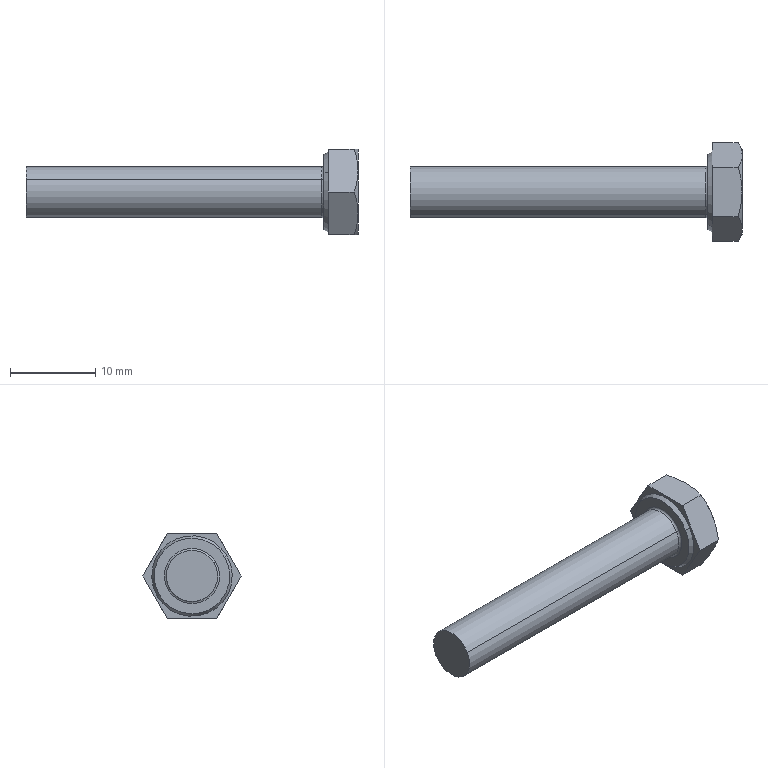Component | SolidWorks | GB_T5782-2016[HexHeadBoltM6_35]-4 | 1 solid | 22 faces | box 39 x 11.55 x 10 mm | volume 1325 mm3 | plane 10 | cone 8 | torus 2 | cylinder 2 | commonest cylinder face diameters 6 x2
build123d program:
from build123d import *

# Parameters (mm, degrees)
BASE_EXTRUDE_DEPTH = 4
FILLET_2_R         = 0.25


with BuildPart() as part:
    # Sketch1 → Base-Extrude (new body)
    with BuildSketch(Plane(origin=(0, 0, 0), x_dir=(0, 0, -1), z_dir=(1, 0, 0))):
        Polygon((5, 2.887), (5, -2.887), (0, -5.774), (-5, -2.887), (-5, 2.887), (0, 5.774), align=None)
    extrude(amount=BASE_EXTRUDE_DEPTH)

    # Sketch2 → Revolve1 (revolve)
    with BuildSketch(Plane.XY, mode=Mode.PRIVATE) as revolve1_sk:
        Polygon((0, 0), (39, 0), (39, 2.134), (39, 3), (21, 3), (0, 3), align=None)
    revolve(revolve1_sk.sketch.rotate(Axis((0, 0, 0), (1, 0, 0)), 90), axis=Axis((0, 0, 0), (1, 0, 0)))

    # Sketch3 → Cut-Revolve1 (revolve, cut)
    with BuildSketch(Plane.XY):
        Polygon((0, 5), (3.333, 10.774), (3.333, 15.774), (-10, 15.774), (-10, 5), align=None)
    revolve(axis=Axis((0, 0, 0), (1, 0, 0)), mode=Mode.SUBTRACT)

    # Sketch4 → Cut-Revolve3 (revolve, cut)
    with BuildSketch(Plane.XY, mode=Mode.PRIVATE) as cut_revolve3_sk:
        Polygon((4, 4.44), (3.5, 4.729), (3.5, 5.774), (4, 5.774), align=None)
    revolve(cut_revolve3_sk.sketch.rotate(Axis((0, 0, 0), (1, 0, 0)), 90), axis=Axis((0, 0, 0), (1, 0, 0)), mode=Mode.SUBTRACT)

    # Fillet 2
    fillet_2_edges = [part.edges().sort_by_distance(p)[0] for p in [
        (4, 0, -3),
    ]]
    fillet(fillet_2_edges, radius=FILLET_2_R)


solid = part.part

# Placed as in the assembly
solid = solid.moved(Location((4, 0, -95), (-180, 0, 180)))
STEP:
#1=COLOUR_RGB('',0.7922,0.8196,0.9333);
#2=FILL_AREA_STYLE_COLOUR('',#1);
#3=FILL_AREA_STYLE('',(#2));
#4=SURFACE_STYLE_FILL_AREA(#3);
#5=SURFACE_SIDE_STYLE('',(#4));
#6=SURFACE_STYLE_USAGE(.BOTH.,#5);
#7=PRESENTATION_STYLE_ASSIGNMENT((#6));
#8=CARTESIAN_POINT('',(-0.009843,-0.1023,-3.681));
#9=VERTEX_POINT('',#8);
#10=CARTESIAN_POINT('',(-0.009843,0.1023,-3.799));
#11=VERTEX_POINT('',#10);
#12=CARTESIAN_POINT('',(-0.009843,0.,-3.74));
#13=DIRECTION('',(-1.,-0.,0.));
#14=DIRECTION('',(-0.,0.866,-0.5));
#15=AXIS2_PLACEMENT_3D('',#12,#13,#14);
#16=CIRCLE('',#15,0.1181);
#17=EDGE_CURVE('',#9,#11,#16,.T.);
#18=ORIENTED_EDGE('',*,*,#17,.F.);
#19=CARTESIAN_POINT('',(0.,-0.1108,-3.676));
#20=VERTEX_POINT('',#19);
#21=CARTESIAN_POINT('',(-0.009843,-0.1108,-3.676));
#22=DIRECTION('',(0.,-0.5,-0.866));
#23=DIRECTION('',(0.,0.866,-0.5));
#24=AXIS2_PLACEMENT_3D('',#21,#22,#23);
#25=CIRCLE('',#24,0.009843);
#26=EDGE_CURVE('',#9,#20,#25,.T.);
#27=ORIENTED_EDGE('',*,*,#26,.T.);
#28=CARTESIAN_POINT('',(0.,0.1108,-3.804));
#29=VERTEX_POINT('',#28);
#30=CARTESIAN_POINT('',(0.,0.,-3.74));
#31=DIRECTION('',(1.,0.,-0.));
#32=DIRECTION('',(-0.,0.866,-0.5));
#33=AXIS2_PLACEMENT_3D('',#30,#31,#32);
#34=CIRCLE('',#33,0.128);
#35=EDGE_CURVE('',#29,#20,#34,.T.);
#36=ORIENTED_EDGE('',*,*,#35,.F.);
#37=CARTESIAN_POINT('',(-0.009843,0.1108,-3.804));
#38=DIRECTION('',(-0.,0.5,0.866));
#39=DIRECTION('',(0.,-0.866,0.5));
#40=AXIS2_PLACEMENT_3D('',#37,#38,#39);
#41=CIRCLE('',#40,0.009843);
#42=EDGE_CURVE('',#11,#29,#41,.T.);
#43=ORIENTED_EDGE('',*,*,#42,.F.);
#44=EDGE_LOOP('',(#18,#27,#36,#43));
#45=FACE_OUTER_BOUND('',#44,.T.);
#46=CARTESIAN_POINT('',(-0.009843,0.,-3.74));
#47=DIRECTION('',(-1.,-0.,0.));
#48=DIRECTION('',(-0.,0.866,-0.5));
#49=AXIS2_PLACEMENT_3D('',#46,#47,#48);
#50=TOROIDAL_SURFACE('',#49,0.128,0.009843);
#51=ADVANCED_FACE('',(#45),#50,.F.);
#52=CARTESIAN_POINT('',(-1.378,-0.1023,-3.681));
#53=VERTEX_POINT('',#52);
#54=CARTESIAN_POINT('',(-1.378,0.1023,-3.799));
#55=VERTEX_POINT('',#54);
#56=CARTESIAN_POINT('',(-1.378,0.,-3.74));
#57=DIRECTION('',(1.,0.,-0.));
#58=DIRECTION('',(0.,-0.866,0.5));
#59=AXIS2_PLACEMENT_3D('',#56,#57,#58);
#60=CIRCLE('',#59,0.1181);
#61=EDGE_CURVE('',#53,#55,#60,.T.);
#62=ORIENTED_EDGE('',*,*,#61,.T.);
#63=CARTESIAN_POINT('',(0.1575,0.1023,-3.799));
#64=DIRECTION('',(1.,0.,-0.));
#65=VECTOR('',#64,39.37);
#66=LINE('',#63,#65);
#67=EDGE_CURVE('',#55,#11,#66,.T.);
#68=ORIENTED_EDGE('',*,*,#67,.T.);
#69=CARTESIAN_POINT('',(-0.009843,0.,-3.74));
#70=DIRECTION('',(-1.,-0.,0.));
#71=DIRECTION('',(-0.,0.866,-0.5));
#72=AXIS2_PLACEMENT_3D('',#69,#70,#71);
#73=CIRCLE('',#72,0.1181);
#74=EDGE_CURVE('',#11,#9,#73,.T.);
#75=ORIENTED_EDGE('',*,*,#74,.T.);
#76=CARTESIAN_POINT('',(0.1575,-0.1023,-3.681));
#77=DIRECTION('',(1.,0.,-0.));
#78=VECTOR('',#77,39.37);
#79=LINE('',#76,#78);
#80=EDGE_CURVE('',#53,#9,#79,.T.);
#81=ORIENTED_EDGE('',*,*,#80,.F.);
#82=EDGE_LOOP('',(#62,#68,#75,#81));
#83=FACE_OUTER_BOUND('',#82,.T.);
#84=CARTESIAN_POINT('',(0.1575,0.,-3.74));
#85=DIRECTION('',(1.,0.,-0.));
#86=DIRECTION('',(0.,-0.866,0.5));
#87=AXIS2_PLACEMENT_3D('',#84,#85,#86);
#88=CYLINDRICAL_SURFACE('',#87,0.1181);
#89=ADVANCED_FACE('',(#83),#88,.T.);
#90=CARTESIAN_POINT('',(0.,-0.1514,-3.653));
#91=VERTEX_POINT('',#90);
#92=CARTESIAN_POINT('',(0.,0.1514,-3.828));
#93=VERTEX_POINT('',#92);
#94=CARTESIAN_POINT('',(0.,0.,-3.74));
#95=DIRECTION('',(1.,0.,-0.));
#96=DIRECTION('',(0.,-0.866,0.5));
#97=AXIS2_PLACEMENT_3D('',#94,#95,#96);
#98=CIRCLE('',#97,0.1748);
#99=EDGE_CURVE('',#91,#93,#98,.T.);
#100=ORIENTED_EDGE('',*,*,#99,.T.);
#101=CARTESIAN_POINT('',(0.01969,0.1612,-3.833));
#102=VERTEX_POINT('',#101);
#103=CARTESIAN_POINT('',(0.01969,0.1612,-3.833));
#104=DIRECTION('',(0.866,0.433,-0.25));
#105=VECTOR('',#104,39.37);
#106=LINE('',#103,#105);
#107=EDGE_CURVE('',#93,#102,#106,.T.);
#108=ORIENTED_EDGE('',*,*,#107,.T.);
#109=CARTESIAN_POINT('',(0.01969,-0.1612,-3.647));
#110=VERTEX_POINT('',#109);
#111=CARTESIAN_POINT('',(0.01969,0.,-3.74));
#112=DIRECTION('',(1.,0.,-0.));
#113=DIRECTION('',(0.,-0.866,0.5));
#114=AXIS2_PLACEMENT_3D('',#111,#112,#113);
#115=CIRCLE('',#114,0.1862);
#116=EDGE_CURVE('',#110,#102,#115,.T.);
#117=ORIENTED_EDGE('',*,*,#116,.F.);
#118=CARTESIAN_POINT('',(0.01969,-0.1612,-3.647));
#119=DIRECTION('',(0.866,-0.433,0.25));
#120=VECTOR('',#119,39.37);
#121=LINE('',#118,#120);
#122=EDGE_CURVE('',#91,#110,#121,.T.);
#123=ORIENTED_EDGE('',*,*,#122,.F.);
#124=EDGE_LOOP('',(#100,#108,#117,#123));
#125=FACE_OUTER_BOUND('',#124,.T.);
#126=CARTESIAN_POINT('',(0.01969,0.,-3.74));
#127=DIRECTION('',(1.,0.,-0.));
#128=DIRECTION('',(0.,-0.866,0.5));
#129=AXIS2_PLACEMENT_3D('',#126,#127,#128);
#130=CONICAL_SURFACE('',#129,0.1862,0.5236);
#131=ADVANCED_FACE('',(#125),#130,.T.);
#132=CARTESIAN_POINT('',(0.01969,0.1137,-3.937));
#133=VERTEX_POINT('',#132);
#134=CARTESIAN_POINT('',(0.01969,-0.1137,-3.937));
#135=VERTEX_POINT('',#134);
#136=CARTESIAN_POINT('',(0.01969,0.1137,-3.937));
#137=DIRECTION('',(0.,-1.,-0.));
#138=VECTOR('',#137,39.37);
#139=LINE('',#136,#138);
#140=EDGE_CURVE('',#133,#135,#139,.T.);
#141=ORIENTED_EDGE('',*,*,#140,.F.);
#142=CARTESIAN_POINT('',(0.1399,0.1137,-3.937));
#143=VERTEX_POINT('',#142);
#144=CARTESIAN_POINT('',(0.,0.1137,-3.937));
#145=DIRECTION('',(1.,0.,-0.));
#146=VECTOR('',#145,39.37);
#147=LINE('',#144,#146);
#148=EDGE_CURVE('',#133,#143,#147,.T.);
#149=ORIENTED_EDGE('',*,*,#148,.T.);
#150=CARTESIAN_POINT('',(0.1575,0.,-3.937));
#151=VERTEX_POINT('',#150);
#152=CARTESIAN_POINT('',(0.1575,0.,-3.937));
#153=CARTESIAN_POINT('',(0.1575,0.009645,-3.937));
#154=CARTESIAN_POINT('',(0.1571,0.01933,-3.937));
#155=CARTESIAN_POINT('',(0.1555,0.0385,-3.937));
#156=CARTESIAN_POINT('',(0.1543,0.04802,-3.937));
#157=CARTESIAN_POINT('',(0.1497,0.07641,-3.937));
#158=CARTESIAN_POINT('',(0.1453,0.09511,-3.937));
#159=CARTESIAN_POINT('',(0.1399,0.1137,-3.937));
#160=B_SPLINE_CURVE_WITH_KNOTS('',3,(#152,#153,#154,#155,#156,#157,#158,#159),.UNSPECIFIED.,.F.,.F.,(4,2,2,4),(0.002921,0.003649,0.004376,0.005831),.UNSPECIFIED.);
#161=EDGE_CURVE('',#151,#143,#160,.T.);
#162=ORIENTED_EDGE('',*,*,#161,.F.);
#163=CARTESIAN_POINT('',(0.1399,-0.1137,-3.937));
#164=VERTEX_POINT('',#163);
#165=CARTESIAN_POINT('',(0.1399,-0.1137,-3.937));
#166=CARTESIAN_POINT('',(0.1506,-0.07647,-3.937));
#167=CARTESIAN_POINT('',(0.1575,-0.03873,-3.937));
#168=CARTESIAN_POINT('',(0.1575,0.,-3.937));
#169=B_SPLINE_CURVE_WITH_KNOTS('',3,(#165,#166,#167,#168),.UNSPECIFIED.,.F.,.F.,(4,4),(0.00000024,0.002921),.UNSPECIFIED.);
#170=EDGE_CURVE('',#164,#151,#169,.T.);
#171=ORIENTED_EDGE('',*,*,#170,.F.);
#172=CARTESIAN_POINT('',(0.,-0.1137,-3.937));
#173=DIRECTION('',(1.,0.,-0.));
#174=VECTOR('',#173,39.37);
#175=LINE('',#172,#174);
#176=EDGE_CURVE('',#135,#164,#175,.T.);
#177=ORIENTED_EDGE('',*,*,#176,.F.);
#178=EDGE_LOOP('',(#141,#149,#162,#171,#177));
#179=FACE_OUTER_BOUND('',#178,.T.);
#180=CARTESIAN_POINT('',(0.,0.1137,-3.937));
#181=DIRECTION('',(0.,-0.,1.));
#182=DIRECTION('',(-0.,1.,0.));
#183=AXIS2_PLACEMENT_3D('',#180,#181,#182);
#184=PLANE('',#183);
#185=ADVANCED_FACE('',(#179),#184,.F.);
#186=CARTESIAN_POINT('',(0.01969,-0.2273,-3.74));
#187=VERTEX_POINT('',#186);
#188=CARTESIAN_POINT('',(0.01969,-0.1137,-3.937));
#189=DIRECTION('',(0.,-0.5,0.866));
#190=VECTOR('',#189,39.37);
#191=LINE('',#188,#190);
#192=EDGE_CURVE('',#135,#187,#191,.T.);
#193=ORIENTED_EDGE('',*,*,#192,.F.);
#194=ORIENTED_EDGE('',*,*,#176,.T.);
#195=CARTESIAN_POINT('',(0.1575,-0.1705,-3.839));
#196=VERTEX_POINT('',#195);
#197=CARTESIAN_POINT('',(0.1575,-0.1705,-3.839));
#198=CARTESIAN_POINT('',(0.1575,-0.1657,-3.847));
#199=CARTESIAN_POINT('',(0.1571,-0.1608,-3.855));
#200=CARTESIAN_POINT('',(0.1555,-0.1512,-3.872));
#201=CARTESIAN_POINT('',(0.1543,-0.1465,-3.88));
#202=CARTESIAN_POINT('',(0.1497,-0.1323,-3.905));
#203=CARTESIAN_POINT('',(0.1453,-0.1229,-3.921));
#204=CARTESIAN_POINT('',(0.1399,-0.1137,-3.937));
#205=B_SPLINE_CURVE_WITH_KNOTS('',3,(#197,#198,#199,#200,#201,#202,#203,#204),.UNSPECIFIED.,.F.,.F.,(4,2,2,4),(0.002921,0.003649,0.004376,0.005831),.UNSPECIFIED.);
#206=EDGE_CURVE('',#196,#164,#205,.T.);
#207=ORIENTED_EDGE('',*,*,#206,.F.);
#208=CARTESIAN_POINT('',(0.1399,-0.2273,-3.74));
#209=VERTEX_POINT('',#208);
#210=CARTESIAN_POINT('',(0.1399,-0.2273,-3.74));
#211=CARTESIAN_POINT('',(0.1506,-0.2087,-3.772));
#212=CARTESIAN_POINT('',(0.1575,-0.1898,-3.805));
#213=CARTESIAN_POINT('',(0.1575,-0.1705,-3.839));
#214=B_SPLINE_CURVE_WITH_KNOTS('',3,(#210,#211,#212,#213),.UNSPECIFIED.,.F.,.F.,(4,4),(0.00000024,0.002921),.UNSPECIFIED.);
#215=EDGE_CURVE('',#209,#196,#214,.T.);
#216=ORIENTED_EDGE('',*,*,#215,.F.);
#217=CARTESIAN_POINT('',(0.,-0.2273,-3.74));
#218=DIRECTION('',(1.,0.,-0.));
#219=VECTOR('',#218,39.37);
#220=LINE('',#217,#219);
#221=EDGE_CURVE('',#187,#209,#220,.T.);
#222=ORIENTED_EDGE('',*,*,#221,.F.);
#223=EDGE_LOOP('',(#193,#194,#207,#216,#222));
#224=FACE_OUTER_BOUND('',#223,.T.);
#225=CARTESIAN_POINT('',(0.,-0.1137,-3.937));
#226=DIRECTION('',(-0.,0.866,0.5));
#227=DIRECTION('',(-0.,0.5,-0.866));
#228=AXIS2_PLACEMENT_3D('',#225,#226,#227);
#229=PLANE('',#228);
#230=ADVANCED_FACE('',(#224),#229,.F.);
#231=CARTESIAN_POINT('',(0.01969,-0.1137,-3.543));
#232=VERTEX_POINT('',#231);
#233=CARTESIAN_POINT('',(0.01969,-0.2273,-3.74));
#234=DIRECTION('',(-0.,0.5,0.866));
#235=VECTOR('',#234,39.37);
#236=LINE('',#233,#235);
#237=EDGE_CURVE('',#187,#232,#236,.T.);
#238=ORIENTED_EDGE('',*,*,#237,.F.);
#239=ORIENTED_EDGE('',*,*,#221,.T.);
#240=CARTESIAN_POINT('',(0.1575,-0.1705,-3.642));
#241=VERTEX_POINT('',#240);
#242=CARTESIAN_POINT('',(0.1575,-0.1705,-3.642));
#243=CARTESIAN_POINT('',(0.1575,-0.1801,-3.658));
#244=CARTESIAN_POINT('',(0.1558,-0.1898,-3.675));
#245=CARTESIAN_POINT('',(0.1496,-0.2088,-3.708));
#246=CARTESIAN_POINT('',(0.1452,-0.2181,-3.724));
#247=CARTESIAN_POINT('',(0.1399,-0.2273,-3.74));
#248=B_SPLINE_CURVE_WITH_KNOTS('',3,(#242,#243,#244,#245,#246,#247),.UNSPECIFIED.,.F.,.F.,(4,2,4),(0.008262,0.009724,0.01119),.UNSPECIFIED.);
#249=EDGE_CURVE('',#241,#209,#248,.T.);
#250=ORIENTED_EDGE('',*,*,#249,.F.);
#251=CARTESIAN_POINT('',(0.1399,-0.1137,-3.543));
#252=VERTEX_POINT('',#251);
#253=CARTESIAN_POINT('',(0.1399,-0.1137,-3.543));
#254=CARTESIAN_POINT('',(0.1452,-0.1229,-3.559));
#255=CARTESIAN_POINT('',(0.1497,-0.1324,-3.576));
#256=CARTESIAN_POINT('',(0.1558,-0.1513,-3.609));
#257=CARTESIAN_POINT('',(0.1575,-0.1609,-3.625));
#258=CARTESIAN_POINT('',(0.1575,-0.1705,-3.642));
#259=B_SPLINE_CURVE_WITH_KNOTS('',3,(#253,#254,#255,#256,#257,#258),.UNSPECIFIED.,.F.,.F.,(4,2,4),(0.00534,0.006801,0.008262),.UNSPECIFIED.);
#260=EDGE_CURVE('',#252,#241,#259,.T.);
#261=ORIENTED_EDGE('',*,*,#260,.F.);
#262=CARTESIAN_POINT('',(0.,-0.1137,-3.543));
#263=DIRECTION('',(1.,0.,-0.));
#264=VECTOR('',#263,39.37);
#265=LINE('',#262,#264);
#266=EDGE_CURVE('',#232,#252,#265,.T.);
#267=ORIENTED_EDGE('',*,*,#266,.F.);
#268=EDGE_LOOP('',(#238,#239,#250,#261,#267));
#269=FACE_OUTER_BOUND('',#268,.T.);
#270=CARTESIAN_POINT('',(0.,-0.2273,-3.74));
#271=DIRECTION('',(-0.,0.866,-0.5));
#272=DIRECTION('',(1.,0.,-0.));
#273=AXIS2_PLACEMENT_3D('',#270,#271,#272);
#274=PLANE('',#273);
#275=ADVANCED_FACE('',(#269),#274,.F.);
#276=CARTESIAN_POINT('',(0.01969,0.1137,-3.543));
#277=VERTEX_POINT('',#276);
#278=CARTESIAN_POINT('',(0.01969,0.1137,-3.543));
#279=DIRECTION('',(-0.,1.,0.));
#280=VECTOR('',#279,39.37);
#281=LINE('',#278,#280);
#282=EDGE_CURVE('',#232,#277,#281,.T.);
#283=ORIENTED_EDGE('',*,*,#282,.F.);
#284=ORIENTED_EDGE('',*,*,#266,.T.);
#285=CARTESIAN_POINT('',(0.1575,0.,-3.543));
#286=VERTEX_POINT('',#285);
#287=CARTESIAN_POINT('',(0.1575,0.,-3.543));
#288=CARTESIAN_POINT('',(0.1575,-0.009645,-3.543));
#289=CARTESIAN_POINT('',(0.1571,-0.01933,-3.543));
#290=CARTESIAN_POINT('',(0.1555,-0.0385,-3.543));
#291=CARTESIAN_POINT('',(0.1543,-0.04802,-3.543));
#292=CARTESIAN_POINT('',(0.1497,-0.07641,-3.543));
#293=CARTESIAN_POINT('',(0.1453,-0.09511,-3.543));
#294=CARTESIAN_POINT('',(0.1399,-0.1137,-3.543));
#295=B_SPLINE_CURVE_WITH_KNOTS('',3,(#287,#288,#289,#290,#291,#292,#293,#294),.UNSPECIFIED.,.F.,.F.,(4,2,2,4),(0.002921,0.003649,0.004376,0.005831),.UNSPECIFIED.);
#296=EDGE_CURVE('',#286,#252,#295,.T.);
#297=ORIENTED_EDGE('',*,*,#296,.F.);
#298=CARTESIAN_POINT('',(0.1399,0.1137,-3.543));
#299=VERTEX_POINT('',#298);
#300=CARTESIAN_POINT('',(0.1399,0.1137,-3.543));
#301=CARTESIAN_POINT('',(0.1506,0.07647,-3.543));
#302=CARTESIAN_POINT('',(0.1575,0.03873,-3.543));
#303=CARTESIAN_POINT('',(0.1575,0.,-3.543));
#304=B_SPLINE_CURVE_WITH_KNOTS('',3,(#300,#301,#302,#303),.UNSPECIFIED.,.F.,.F.,(4,4),(0.00000024,0.002921),.UNSPECIFIED.);
#305=EDGE_CURVE('',#299,#286,#304,.T.);
#306=ORIENTED_EDGE('',*,*,#305,.F.);
#307=CARTESIAN_POINT('',(0.,0.1137,-3.543));
#308=DIRECTION('',(1.,0.,-0.));
#309=VECTOR('',#308,39.37);
#310=LINE('',#307,#309);
#311=EDGE_CURVE('',#277,#299,#310,.T.);
#312=ORIENTED_EDGE('',*,*,#311,.F.);
#313=EDGE_LOOP('',(#283,#284,#297,#306,#312));
#314=FACE_OUTER_BOUND('',#313,.T.);
#315=CARTESIAN_POINT('',(0.,0.1137,-3.543));
#316=DIRECTION('',(-0.,0.,-1.));
#317=DIRECTION('',(0.,-1.,-0.));
#318=AXIS2_PLACEMENT_3D('',#315,#316,#317);
#319=PLANE('',#318);
#320=ADVANCED_FACE('',(#314),#319,.F.);
#321=CARTESIAN_POINT('',(0.01969,0.2273,-3.74));
#322=VERTEX_POINT('',#321);
#323=CARTESIAN_POINT('',(0.01969,0.2273,-3.74));
#324=DIRECTION('',(-0.,0.5,-0.866));
#325=VECTOR('',#324,39.37);
#326=LINE('',#323,#325);
#327=EDGE_CURVE('',#277,#322,#326,.T.);
#328=ORIENTED_EDGE('',*,*,#327,.F.);
#329=ORIENTED_EDGE('',*,*,#311,.T.);
#330=CARTESIAN_POINT('',(0.1575,0.1705,-3.642));
#331=VERTEX_POINT('',#330);
#332=CARTESIAN_POINT('',(0.1575,0.1705,-3.642));
#333=CARTESIAN_POINT('',(0.1575,0.1657,-3.633));
#334=CARTESIAN_POINT('',(0.1571,0.1608,-3.625));
#335=CARTESIAN_POINT('',(0.1555,0.1512,-3.608));
#336=CARTESIAN_POINT('',(0.1543,0.1465,-3.6));
#337=CARTESIAN_POINT('',(0.1497,0.1323,-3.576));
#338=CARTESIAN_POINT('',(0.1453,0.1229,-3.559));
#339=CARTESIAN_POINT('',(0.1399,0.1137,-3.543));
#340=B_SPLINE_CURVE_WITH_KNOTS('',3,(#332,#333,#334,#335,#336,#337,#338,#339),.UNSPECIFIED.,.F.,.F.,(4,2,2,4),(0.002921,0.003649,0.004376,0.005831),.UNSPECIFIED.);
#341=EDGE_CURVE('',#331,#299,#340,.T.);
#342=ORIENTED_EDGE('',*,*,#341,.F.);
#343=CARTESIAN_POINT('',(0.1399,0.2273,-3.74));
#344=VERTEX_POINT('',#343);
#345=CARTESIAN_POINT('',(0.1399,0.2273,-3.74));
#346=CARTESIAN_POINT('',(0.1506,0.2087,-3.708));
#347=CARTESIAN_POINT('',(0.1575,0.1898,-3.675));
#348=CARTESIAN_POINT('',(0.1575,0.1705,-3.642));
#349=B_SPLINE_CURVE_WITH_KNOTS('',3,(#345,#346,#347,#348),.UNSPECIFIED.,.F.,.F.,(4,4),(0.00000024,0.002921),.UNSPECIFIED.);
#350=EDGE_CURVE('',#344,#331,#349,.T.);
#351=ORIENTED_EDGE('',*,*,#350,.F.);
#352=CARTESIAN_POINT('',(0.,0.2273,-3.74));
#353=DIRECTION('',(1.,0.,-0.));
#354=VECTOR('',#353,39.37);
#355=LINE('',#352,#354);
#356=EDGE_CURVE('',#322,#344,#355,.T.);
#357=ORIENTED_EDGE('',*,*,#356,.F.);
#358=EDGE_LOOP('',(#328,#329,#342,#351,#357));
#359=FACE_OUTER_BOUND('',#358,.T.);
#360=CARTESIAN_POINT('',(0.,0.2273,-3.74));
#361=DIRECTION('',(0.,-0.866,-0.5));
#362=DIRECTION('',(0.,-0.5,0.866));
#363=AXIS2_PLACEMENT_3D('',#360,#361,#362);
#364=PLANE('',#363);
#365=ADVANCED_FACE('',(#359),#364,.F.);
#366=CARTESIAN_POINT('',(0.01969,0.1137,-3.937));
#367=DIRECTION('',(0.,-0.5,-0.866));
#368=VECTOR('',#367,39.37);
#369=LINE('',#366,#368);
#370=EDGE_CURVE('',#322,#133,#369,.T.);
#371=ORIENTED_EDGE('',*,*,#370,.F.);
#372=ORIENTED_EDGE('',*,*,#356,.T.);
#373=CARTESIAN_POINT('',(0.1575,0.1705,-3.839));
#374=VERTEX_POINT('',#373);
#375=CARTESIAN_POINT('',(0.1575,0.1705,-3.839));
#376=CARTESIAN_POINT('',(0.1575,0.1801,-3.822));
#377=CARTESIAN_POINT('',(0.1558,0.1896,-3.805));
#378=CARTESIAN_POINT('',(0.1497,0.2086,-3.773));
#379=CARTESIAN_POINT('',(0.1452,0.2181,-3.756));
#380=CARTESIAN_POINT('',(0.1399,0.2273,-3.74));
#381=B_SPLINE_CURVE_WITH_KNOTS('',3,(#375,#376,#377,#378,#379,#380),.UNSPECIFIED.,.F.,.F.,(4,2,4),(0.01799,0.01945,0.02091),.UNSPECIFIED.);
#382=EDGE_CURVE('',#374,#344,#381,.T.);
#383=ORIENTED_EDGE('',*,*,#382,.F.);
#384=CARTESIAN_POINT('',(0.1399,0.1137,-3.937));
#385=CARTESIAN_POINT('',(0.1452,0.1228,-3.921));
#386=CARTESIAN_POINT('',(0.1496,0.1322,-3.905));
#387=CARTESIAN_POINT('',(0.1558,0.1511,-3.872));
#388=CARTESIAN_POINT('',(0.1575,0.1609,-3.855));
#389=CARTESIAN_POINT('',(0.1575,0.1705,-3.839));
#390=B_SPLINE_CURVE_WITH_KNOTS('',3,(#384,#385,#386,#387,#388,#389),.UNSPECIFIED.,.F.,.F.,(4,2,4),(0.01507,0.01653,0.01799),.UNSPECIFIED.);
#391=EDGE_CURVE('',#143,#374,#390,.T.);
#392=ORIENTED_EDGE('',*,*,#391,.F.);
#393=ORIENTED_EDGE('',*,*,#148,.F.);
#394=EDGE_LOOP('',(#371,#372,#383,#392,#393));
#395=FACE_OUTER_BOUND('',#394,.T.);
#396=CARTESIAN_POINT('',(0.,0.1137,-3.937));
#397=DIRECTION('',(0.,-0.866,0.5));
#398=DIRECTION('',(-0.,0.5,0.866));
#399=AXIS2_PLACEMENT_3D('',#396,#397,#398);
#400=PLANE('',#399);
#401=ADVANCED_FACE('',(#395),#400,.F.);
#402=ORIENTED_EDGE('',*,*,#350,.T.);
#403=CARTESIAN_POINT('',(0.1575,0.,-3.74));
#404=DIRECTION('',(-1.,-0.,0.));
#405=DIRECTION('',(-0.,0.866,-0.5));
#406=AXIS2_PLACEMENT_3D('',#403,#404,#405);
#407=CIRCLE('',#406,0.1969);
#408=EDGE_CURVE('',#331,#374,#407,.T.);
#409=ORIENTED_EDGE('',*,*,#408,.T.);
#410=ORIENTED_EDGE('',*,*,#382,.T.);
#411=EDGE_LOOP('',(#402,#409,#410));
#412=FACE_OUTER_BOUND('',#411,.T.);
#413=CARTESIAN_POINT('',(0.1575,0.,-3.74));
#414=DIRECTION('',(-1.,-0.,0.));
#415=DIRECTION('',(-0.,0.866,-0.5));
#416=AXIS2_PLACEMENT_3D('',#413,#414,#415);
#417=CONICAL_SURFACE('',#416,0.1969,1.047);
#418=ADVANCED_FACE('',(#412),#417,.T.);
#419=ORIENTED_EDGE('',*,*,#305,.T.);
#420=CARTESIAN_POINT('',(0.1575,0.,-3.74));
#421=DIRECTION('',(-1.,-0.,0.));
#422=DIRECTION('',(-0.,0.866,-0.5));
#423=AXIS2_PLACEMENT_3D('',#420,#421,#422);
#424=CIRCLE('',#423,0.1969);
#425=EDGE_CURVE('',#286,#331,#424,.T.);
#426=ORIENTED_EDGE('',*,*,#425,.T.);
#427=ORIENTED_EDGE('',*,*,#341,.T.);
#428=EDGE_LOOP('',(#419,#426,#427));
#429=FACE_OUTER_BOUND('',#428,.T.);
#430=CARTESIAN_POINT('',(0.1575,0.,-3.74));
#431=DIRECTION('',(-1.,-0.,0.));
#432=DIRECTION('',(-0.,0.866,-0.5));
#433=AXIS2_PLACEMENT_3D('',#430,#431,#432);
#434=CONICAL_SURFACE('',#433,0.1969,1.047);
#435=ADVANCED_FACE('',(#429),#434,.T.);
#436=ORIENTED_EDGE('',*,*,#260,.T.);
#437=CARTESIAN_POINT('',(0.1575,0.,-3.74));
#438=DIRECTION('',(-1.,-0.,0.));
#439=DIRECTION('',(-0.,0.866,-0.5));
#440=AXIS2_PLACEMENT_3D('',#437,#438,#439);
#441=CIRCLE('',#440,0.1969);
#442=EDGE_CURVE('',#241,#286,#441,.T.);
#443=ORIENTED_EDGE('',*,*,#442,.T.);
#444=ORIENTED_EDGE('',*,*,#296,.T.);
#445=EDGE_LOOP('',(#436,#443,#444));
#446=FACE_OUTER_BOUND('',#445,.T.);
#447=CARTESIAN_POINT('',(0.1575,0.,-3.74));
#448=DIRECTION('',(-1.,-0.,0.));
#449=DIRECTION('',(-0.,0.866,-0.5));
#450=AXIS2_PLACEMENT_3D('',#447,#448,#449);
#451=CONICAL_SURFACE('',#450,0.1969,1.047);
#452=ADVANCED_FACE('',(#446),#451,.T.);
#453=ORIENTED_EDGE('',*,*,#249,.T.);
#454=ORIENTED_EDGE('',*,*,#215,.T.);
#455=CARTESIAN_POINT('',(0.1575,0.,-3.74));
#456=DIRECTION('',(1.,0.,-0.));
#457=DIRECTION('',(0.,-0.866,0.5));
#458=AXIS2_PLACEMENT_3D('',#455,#456,#457);
#459=CIRCLE('',#458,0.1969);
#460=EDGE_CURVE('',#241,#196,#459,.T.);
#461=ORIENTED_EDGE('',*,*,#460,.F.);
#462=EDGE_LOOP('',(#453,#454,#461));
#463=FACE_OUTER_BOUND('',#462,.T.);
#464=CARTESIAN_POINT('',(0.1575,0.,-3.74));
#465=DIRECTION('',(-1.,-0.,0.));
#466=DIRECTION('',(-0.,0.866,-0.5));
#467=AXIS2_PLACEMENT_3D('',#464,#465,#466);
#468=CONICAL_SURFACE('',#467,0.1969,1.047);
#469=ADVANCED_FACE('',(#463),#468,.T.);
#470=ORIENTED_EDGE('',*,*,#206,.T.);
#471=ORIENTED_EDGE('',*,*,#170,.T.);
#472=CARTESIAN_POINT('',(0.1575,0.,-3.74));
#473=DIRECTION('',(-1.,-0.,0.));
#474=DIRECTION('',(-0.,0.866,-0.5));
#475=AXIS2_PLACEMENT_3D('',#472,#473,#474);
#476=CIRCLE('',#475,0.1969);
#477=EDGE_CURVE('',#151,#196,#476,.T.);
#478=ORIENTED_EDGE('',*,*,#477,.T.);
#479=EDGE_LOOP('',(#470,#471,#478));
#480=FACE_OUTER_BOUND('',#479,.T.);
#481=CARTESIAN_POINT('',(0.1575,0.,-3.74));
#482=DIRECTION('',(-1.,-0.,0.));
#483=DIRECTION('',(-0.,0.866,-0.5));
#484=AXIS2_PLACEMENT_3D('',#481,#482,#483);
#485=CONICAL_SURFACE('',#484,0.1969,1.047);
#486=ADVANCED_FACE('',(#480),#485,.T.);
#487=ORIENTED_EDGE('',*,*,#161,.T.);
#488=ORIENTED_EDGE('',*,*,#391,.T.);
#489=CARTESIAN_POINT('',(0.1575,0.,-3.74));
#490=DIRECTION('',(-1.,-0.,0.));
#491=DIRECTION('',(-0.,0.866,-0.5));
#492=AXIS2_PLACEMENT_3D('',#489,#490,#491);
#493=CIRCLE('',#492,0.1969);
#494=EDGE_CURVE('',#374,#151,#493,.T.);
#495=ORIENTED_EDGE('',*,*,#494,.T.);
#496=EDGE_LOOP('',(#487,#488,#495));
#497=FACE_OUTER_BOUND('',#496,.T.);
#498=CARTESIAN_POINT('',(0.1575,0.,-3.74));
#499=DIRECTION('',(-1.,-0.,0.));
#500=DIRECTION('',(-0.,0.866,-0.5));
#501=AXIS2_PLACEMENT_3D('',#498,#499,#500);
#502=CONICAL_SURFACE('',#501,0.1969,1.047);
#503=ADVANCED_FACE('',(#497),#502,.T.);
#504=ORIENTED_EDGE('',*,*,#494,.F.);
#505=ORIENTED_EDGE('',*,*,#408,.F.);
#506=ORIENTED_EDGE('',*,*,#425,.F.);
#507=ORIENTED_EDGE('',*,*,#442,.F.);
#508=ORIENTED_EDGE('',*,*,#460,.T.);
#509=ORIENTED_EDGE('',*,*,#477,.F.);
#510=EDGE_LOOP('',(#504,#505,#506,#507,#508,#509));
#511=FACE_OUTER_BOUND('',#510,.T.);
#512=CARTESIAN_POINT('',(0.1575,-0.1137,-3.937));
#513=DIRECTION('',(-1.,-0.,0.));
#514=DIRECTION('',(-0.,0.866,-0.5));
#515=AXIS2_PLACEMENT_3D('',#512,#513,#514);
#516=PLANE('',#515);
#517=ADVANCED_FACE('',(#511),#516,.F.);
#518=ORIENTED_EDGE('',*,*,#116,.T.);
#519=CARTESIAN_POINT('',(0.01969,0.,-3.74));
#520=DIRECTION('',(1.,0.,-0.));
#521=DIRECTION('',(0.,-0.866,0.5));
#522=AXIS2_PLACEMENT_3D('',#519,#520,#521);
#523=CIRCLE('',#522,0.1862);
#524=EDGE_CURVE('',#102,#110,#523,.T.);
#525=ORIENTED_EDGE('',*,*,#524,.T.);
#526=EDGE_LOOP('',(#518,#525));
#527=FACE_BOUND('',#526,.T.);
#528=ORIENTED_EDGE('',*,*,#140,.T.);
#529=ORIENTED_EDGE('',*,*,#192,.T.);
#530=ORIENTED_EDGE('',*,*,#237,.T.);
#531=ORIENTED_EDGE('',*,*,#282,.T.);
#532=ORIENTED_EDGE('',*,*,#327,.T.);
#533=ORIENTED_EDGE('',*,*,#370,.T.);
#534=EDGE_LOOP('',(#528,#529,#530,#531,#532,#533));
#535=FACE_OUTER_BOUND('',#534,.T.);
#536=CARTESIAN_POINT('',(0.01969,-0.09308,-3.901));
#537=DIRECTION('',(-1.,-0.,0.));
#538=DIRECTION('',(-0.,0.866,-0.5));
#539=AXIS2_PLACEMENT_3D('',#536,#537,#538);
#540=PLANE('',#539);
#541=ADVANCED_FACE('',(#527,#535),#540,.T.);
#542=ORIENTED_EDGE('',*,*,#107,.F.);
#543=CARTESIAN_POINT('',(0.,0.,-3.74));
#544=DIRECTION('',(1.,0.,-0.));
#545=DIRECTION('',(0.,-0.866,0.5));
#546=AXIS2_PLACEMENT_3D('',#543,#544,#545);
#547=CIRCLE('',#546,0.1748);
#548=EDGE_CURVE('',#93,#91,#547,.T.);
#549=ORIENTED_EDGE('',*,*,#548,.T.);
#550=ORIENTED_EDGE('',*,*,#122,.T.);
#551=ORIENTED_EDGE('',*,*,#524,.F.);
#552=EDGE_LOOP('',(#542,#549,#550,#551));
#553=FACE_OUTER_BOUND('',#552,.T.);
#554=CARTESIAN_POINT('',(0.01969,0.,-3.74));
#555=DIRECTION('',(1.,0.,-0.));
#556=DIRECTION('',(0.,-0.866,0.5));
#557=AXIS2_PLACEMENT_3D('',#554,#555,#556);
#558=CONICAL_SURFACE('',#557,0.1862,0.5236);
#559=ADVANCED_FACE('',(#553),#558,.T.);
#560=ORIENTED_EDGE('',*,*,#61,.F.);
#561=CARTESIAN_POINT('',(-1.378,0.,-3.74));
#562=DIRECTION('',(1.,0.,-0.));
#563=DIRECTION('',(0.,-0.866,0.5));
#564=AXIS2_PLACEMENT_3D('',#561,#562,#563);
#565=CIRCLE('',#564,0.1181);
#566=EDGE_CURVE('',#55,#53,#565,.T.);
#567=ORIENTED_EDGE('',*,*,#566,.F.);
#568=EDGE_LOOP('',(#560,#567));
#569=FACE_OUTER_BOUND('',#568,.T.);
#570=CARTESIAN_POINT('',(-1.378,0.,-3.74));
#571=DIRECTION('',(1.,0.,-0.));
#572=DIRECTION('',(0.,-0.866,0.5));
#573=AXIS2_PLACEMENT_3D('',#570,#571,#572);
#574=PLANE('',#573);
#575=ADVANCED_FACE('',(#569),#574,.F.);
#576=ORIENTED_EDGE('',*,*,#67,.F.);
#577=ORIENTED_EDGE('',*,*,#566,.T.);
#578=ORIENTED_EDGE('',*,*,#80,.T.);
#579=ORIENTED_EDGE('',*,*,#17,.T.);
#580=EDGE_LOOP('',(#576,#577,#578,#579));
#581=FACE_OUTER_BOUND('',#580,.T.);
#582=CARTESIAN_POINT('',(0.1575,0.,-3.74));
#583=DIRECTION('',(1.,0.,-0.));
#584=DIRECTION('',(0.,-0.866,0.5));
#585=AXIS2_PLACEMENT_3D('',#582,#583,#584);
#586=CYLINDRICAL_SURFACE('',#585,0.1181);
#587=ADVANCED_FACE('',(#581),#586,.T.);
#588=ORIENTED_EDGE('',*,*,#35,.T.);
#589=CARTESIAN_POINT('',(0.,0.,-3.74));
#590=DIRECTION('',(1.,0.,-0.));
#591=DIRECTION('',(-0.,0.866,-0.5));
#592=AXIS2_PLACEMENT_3D('',#589,#590,#591);
#593=CIRCLE('',#592,0.128);
#594=EDGE_CURVE('',#20,#29,#593,.T.);
#595=ORIENTED_EDGE('',*,*,#594,.T.);
#596=EDGE_LOOP('',(#588,#595));
#597=FACE_BOUND('',#596,.T.);
#598=ORIENTED_EDGE('',*,*,#99,.F.);
#599=ORIENTED_EDGE('',*,*,#548,.F.);
#600=EDGE_LOOP('',(#598,#599));
#601=FACE_OUTER_BOUND('',#600,.T.);
#602=CARTESIAN_POINT('',(0.,-0.1137,-3.937));
#603=DIRECTION('',(-1.,-0.,0.));
#604=DIRECTION('',(-0.,0.866,-0.5));
#605=AXIS2_PLACEMENT_3D('',#602,#603,#604);
#606=PLANE('',#605);
#607=ADVANCED_FACE('',(#597,#601),#606,.T.);
#608=ORIENTED_EDGE('',*,*,#26,.F.);
#609=ORIENTED_EDGE('',*,*,#74,.F.);
#610=ORIENTED_EDGE('',*,*,#42,.T.);
#611=ORIENTED_EDGE('',*,*,#594,.F.);
#612=EDGE_LOOP('',(#608,#609,#610,#611));
#613=FACE_OUTER_BOUND('',#612,.T.);
#614=CARTESIAN_POINT('',(-0.009843,0.,-3.74));
#615=DIRECTION('',(-1.,-0.,0.));
#616=DIRECTION('',(-0.,0.866,-0.5));
#617=AXIS2_PLACEMENT_3D('',#614,#615,#616);
#618=TOROIDAL_SURFACE('',#617,0.128,0.009843);
#619=ADVANCED_FACE('',(#613),#618,.F.);
#620=CLOSED_SHELL('',(#51,#89,#131,#185,#230,#275,#320,#365,#401,#418,#435,#452,#469,#486,#503,#517,#541,#559,#575,#587,#607,#619));
#621=MANIFOLD_SOLID_BREP('',#620);
#622=STYLED_ITEM('',(#7),#621);
#623=PRESENTATION_LAYER_ASSIGNMENT('','',(#622));
#624=(LENGTH_UNIT()NAMED_UNIT(*)SI_UNIT($,.METRE.));
#625=LENGTH_MEASURE_WITH_UNIT(LENGTH_MEASURE(0.0254),#624);
#626=DIMENSIONAL_EXPONENTS(1.,0.,0.,0.,0.,0.,0.);
#627=(CONVERSION_BASED_UNIT('',#625)LENGTH_UNIT()NAMED_UNIT(#626));
#628=UNCERTAINTY_MEASURE_WITH_UNIT(LENGTH_MEASURE(0.00001),#627,'','');
#629=(NAMED_UNIT(*)PLANE_ANGLE_UNIT()SI_UNIT($,.RADIAN.));
#630=(NAMED_UNIT(*)SI_UNIT($,.STERADIAN.)SOLID_ANGLE_UNIT());
#631=(GEOMETRIC_REPRESENTATION_CONTEXT(3)GLOBAL_UNCERTAINTY_ASSIGNED_CONTEXT((#628))GLOBAL_UNIT_ASSIGNED_CONTEXT((#627,#629,#630))REPRESENTATION_CONTEXT('',''));
#632=MECHANICAL_DESIGN_GEOMETRIC_PRESENTATION_REPRESENTATION('',(#622),#631);
#633=CARTESIAN_POINT('',(0.,0.,0.));
#634=DIRECTION('',(0.,0.,1.));
#635=DIRECTION('',(1.,0.,0.));
#636=AXIS2_PLACEMENT_3D('',#633,#634,#635);
#637=(LENGTH_UNIT()NAMED_UNIT(*)SI_UNIT($,.METRE.));
#638=LENGTH_MEASURE_WITH_UNIT(LENGTH_MEASURE(0.0254),#637);
#639=DIMENSIONAL_EXPONENTS(1.,0.,0.,0.,0.,0.,0.);
#640=(CONVERSION_BASED_UNIT('',#638)LENGTH_UNIT()NAMED_UNIT(#639));
#641=UNCERTAINTY_MEASURE_WITH_UNIT(LENGTH_MEASURE(0.00001),#640,'','');
#642=(NAMED_UNIT(*)PLANE_ANGLE_UNIT()SI_UNIT($,.RADIAN.));
#643=(NAMED_UNIT(*)SI_UNIT($,.STERADIAN.)SOLID_ANGLE_UNIT());
#644=(GEOMETRIC_REPRESENTATION_CONTEXT(3)GLOBAL_UNCERTAINTY_ASSIGNED_CONTEXT((#641))GLOBAL_UNIT_ASSIGNED_CONTEXT((#640,#642,#643))REPRESENTATION_CONTEXT('',''));
#645=ADVANCED_BREP_SHAPE_REPRESENTATION('',(#621,#636),#644);